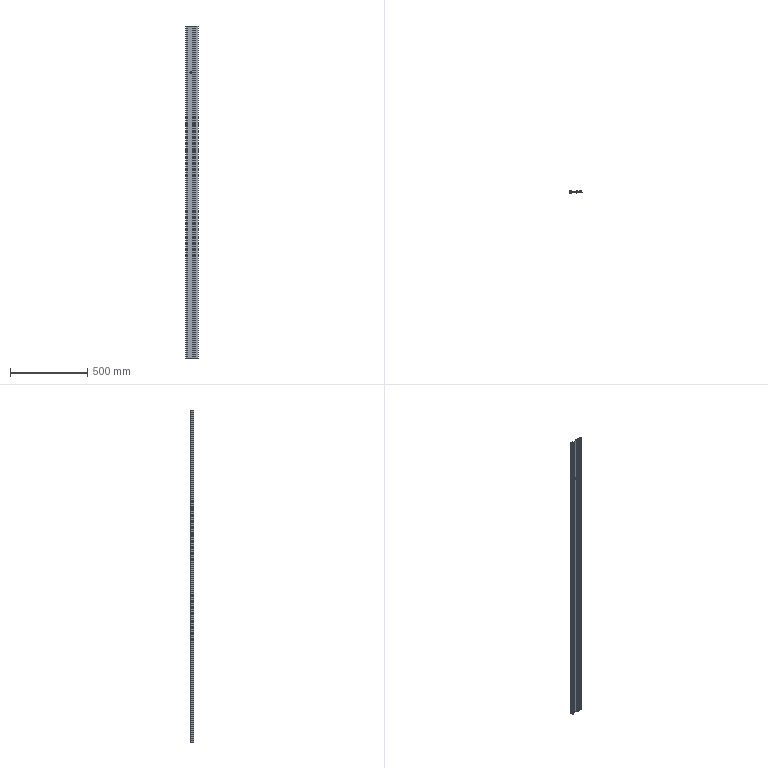Component | SolidWorks | RackArm-3 | 1 solid | 64 faces | box 80.2 x 22 x 2150 mm | volume 697523 mm3 | plane 57 | cylinder 7 | commonest cylinder face diameters 2 x3 11.2 x2 4 x2
build123d program:
from build123d import *

# Parameters (mm, degrees)
BOSS_EXTRUDE1_DEPTH = 2150
SKETCH2_R           = 5.6
CUT_EXTRUDE1_DEPTH  = 10


with BuildPart() as part:
    # Sketch1 → Boss-Extrude1 (new body)
    with BuildSketch(Plane.XY):
        with BuildLine():
            Line((17.75, 8.5), (17.5, 8.3))
            Line((17.5, 8.3), (17.25, 8.5))
            Line((17.25, 8.5), (0, 8.5))
            Line((0, 8.5), (0, 14.9))
            Line((0, 14.9), (-7, 14.9))
            Line((-7, 14.9), (-7, 17.4))
            ThreePointArc((-7, 17.4), (-8.414, 16.814), (-9, 15.4))
            Line((-9, 15.4), (-9, 10.4))
            Line((-9, 10.4), (-7, 10.4))
            Line((-7, 10.4), (-7, 12.7))
            Line((-7, 12.7), (-2, 12.7))
            Line((-2, 12.7), (-2, 7.75))
            Line((-2, 7.75), (-1.75, 7.5))
            Line((-1.75, 7.5), (-2, 7.25))
            Line((-2, 7.25), (-2, 2.2))
            Line((-2, 2.2), (-7, 2.2))
            Line((-7, 2.2), (-7, 4.5))
            Line((-7, 4.5), (-9, 4.5))
            Line((-9, 4.5), (-9, -0.5))
            ThreePointArc((-9, -0.5), (-8.414, -1.914), (-7, -2.5))
            Line((-7, -2.5), (-7, 0))
            Line((-7, 0), (0, 0))
            Line((0, 0), (0, 6.5))
            Line((0, 6.5), (35, 6.5))
            Line((35, 6.5), (35, -2.5))
            ThreePointArc((35, -2.5), (35.293, -3.207), (36, -3.5))
            ThreePointArc((36, -3.5), (36.707, -3.207), (37, -2.5))
            Line((37, -2.5), (37, 6.5))
            Line((37, 6.5), (44, 6.5))
            Line((44, 6.5), (44, 3.5))
            Line((44, 3.5), (48.3, 3.5))
            Line((48.3, 3.5), (48.3, 5.5))
            Line((48.3, 5.5), (46.2, 5.5))
            Line((46.2, 5.5), (46.2, 10.5))
            Line((46.2, 10.5), (56.9, 10.5))
            Line((56.9, 10.5), (56.9, 5.5))
            Line((56.9, 5.5), (54.8, 5.5))
            Line((54.8, 5.5), (54.8, 3.5))
            Line((54.8, 3.5), (70.2, 3.5))
            ThreePointArc((70.2, 3.5), (70.907, 3.793), (71.2, 4.5))
            ThreePointArc((71.2, 4.5), (70.907, 5.207), (70.2, 5.5))
            Line((70.2, 5.5), (67.588, 5.901))
            Line((67.588, 5.901), (67.5, 5.2))
            Line((67.5, 5.2), (62.5, 6))
            Line((62.5, 6), (59, 6))
            Line((59, 6), (59, 10))
            Line((59, 10), (62.5, 10))
            Line((62.5, 10), (67.5, 10.8))
            Line((67.5, 10.8), (67.6, 10))
            Line((67.6, 10), (69.5, 10))
            Line((69.5, 10), (69.5, 12.5))
            Line((69.5, 12.5), (51.8, 12.5))
            Line((51.8, 12.5), (51.55, 12.3))
            Line((51.55, 12.3), (51.3, 12.5))
            Line((51.3, 12.5), (44, 12.5))
            Line((44, 12.5), (44, 8.5))
            Line((44, 8.5), (37, 8.5))
            Line((37, 8.5), (37, 17.5))
            ThreePointArc((37, 17.5), (36.707, 18.207), (36, 18.5))
            ThreePointArc((36, 18.5), (35.293, 18.207), (35, 17.5))
            Line((35, 17.5), (35, 8.5))
            Line((35, 8.5), (17.75, 8.5))
        make_face()
    extrude(amount=BOSS_EXTRUDE1_DEPTH)

    # Sketch2 → Cut-Extrude1 (cut)
    with BuildSketch(Plane.XZ.offset(-6.5)):
        with Locations(Location((23, 1850, 0), (0, 0, 270))):
            Circle(SKETCH2_R)
    extrude(amount=-CUT_EXTRUDE1_DEPTH, mode=Mode.SUBTRACT)


solid = part.part

# Placed as in the assembly
solid = solid.moved(Location((-36.793, 494.747, -258.936), (0, 0, 0)))